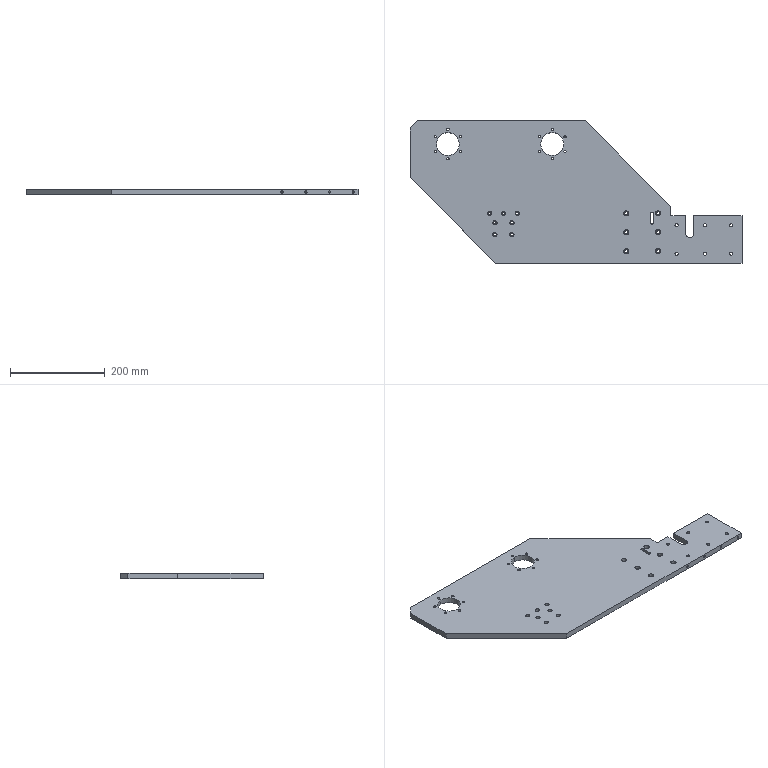Component | SolidWorks | LD101-02--Q1012-Q1-2-5 | 1 solid | 176 faces | box 700 x 300 x 12 mm | volume 1696516 mm3 | cylinder 125 | plane 35 | cone 16 | commonest cylinder face diameters 5 x32 11 x24 6.6 x24 5.5 x17 9 x14 4.2 x8 48.2 x4 17 x2 | material AL6061
build123d program:
from build123d import *

# Parameters (mm, degrees)
SKETCH1_W                                           = 700
SKETCH1_H                                           = 300
BOSS_EXTRUDE1_DEPTH                                 = 6
SKETCH2_W                                           = 150
SKETCH2_H                                           = 200
CUT_EXTRUDE1_DEPTH                                  = 381.978
CUT_EXTRUDE4_DEPTH                                  = 381.978
HOLE_SIZE_ACCORDING_TO_TYPE0_OF_HEXAGON_D           = 6.6
HOLE_SIZE_ACCORDING_TO_TYPE0_OF_HEXAGON_CBORE_D     = 11
HOLE_SIZE_ACCORDING_TO_TYPE0_OF_HEXAGON_CBORE_DEPTH = 6.8
M6_TAPPED_HOLE2_D                                   = 5
M6_TAPPED_HOLE2_DEPTH                               = 20
M6_TAPPED_HOLE2_TIP                                 = 1.502
CUT_EXTRUDE6_DEPTH                                  = 381.978
CUT_EXTRUDE7_DEPTH                                  = 381.978
HOLE_SIZE_FOR_HEX_SOCKET_HEAD_CAP_SCRE_D            = 6.6
HOLE_SIZE_FOR_HEX_SOCKET_HEAD_CAP_SCRE_CBORE_D      = 11
HOLE_SIZE_FOR_HEX_SOCKET_HEAD_CAP_SCRE_CBORE_DEPTH  = 6.8
CHAMFER1_SIZE                                       = 15
SKETCH18_R                                          = 24.1
CUT_EXTRUDE8_DEPTH                                  = 381.978
HOLE_SIZE_ACCORDING_TO_HEXAGON_SOCKET_H_D           = 5.5
HOLE_SIZE_ACCORDING_TO_HEXAGON_SOCKET_H_CBORE_D     = 9
HOLE_SIZE_ACCORDING_TO_HEXAGON_SOCKET_H_CBORE_DEPTH = 5.7
M5_TAPPED_HOLE1_D                                   = 4.2
M5_TAPPED_HOLE1_DEPTH                               = 16
M5_TAPPED_HOLE1_TIP                                 = 1.262
M6_TAPPED_HOLE3_D                                   = 5


with BuildPart() as part:
    # Sketch1 → Boss-Extrude1 (new, symmetric)
    with BuildSketch(Plane(origin=(0, 0, 0), x_dir=(1, 0, 0), z_dir=(0, 1, 0))):
        Rectangle(SKETCH1_W, SKETCH1_H)
    extrude(amount=BOSS_EXTRUDE1_DEPTH, both=True)

    # Sketch2 → Cut-Extrude1 (cut, through all)
    with BuildSketch(Plane.XZ.offset(6)):
        with Locations((275, 50)):
            Rectangle(SKETCH2_W, SKETCH2_H)
    extrude(amount=-CUT_EXTRUDE1_DEPTH, mode=Mode.SUBTRACT)

    # Sketch5 → Cut-Extrude4 (cut, through all)
    with BuildSketch(Plane.XZ.offset(6)):
        with BuildLine():
            Line((157.25, -65), (157.25, -45))
            ThreePointArc((157.25, -45), (160, -42.25), (162.75, -45))
            Line((162.75, -45), (162.75, -65))
            ThreePointArc((162.75, -65), (160, -67.75), (157.25, -65))
        make_face()
    extrude(amount=-CUT_EXTRUDE4_DEPTH, mode=Mode.SUBTRACT)

    # Hole Size_according to_Type0 of Hexagon (through all)
    with Locations(Plane(origin=(0, 6, 0), x_dir=(1, 0, 0), z_dir=(0, 1, 0))):
        with Locations((327, 70), (272, 70), (212, 70), (212, 130), (327, 130), (272, 130)):
            CounterBoreHole(HOLE_SIZE_ACCORDING_TO_TYPE0_OF_HEXAGON_D / 2, HOLE_SIZE_ACCORDING_TO_TYPE0_OF_HEXAGON_CBORE_D / 2, HOLE_SIZE_ACCORDING_TO_TYPE0_OF_HEXAGON_CBORE_DEPTH)

    # M6 Tapped Hole2
    with Locations(Plane(origin=(0, 0, -150), x_dir=(-1, 0, 0), z_dir=(0, 0, -1))):
        with Locations((-340, 0), (-290, 0), (-240, 0), (-190, 0)):
            Hole(M6_TAPPED_HOLE2_D / 2, depth=M6_TAPPED_HOLE2_DEPTH)
            with Locations((0, 0, -(M6_TAPPED_HOLE2_DEPTH + M6_TAPPED_HOLE2_TIP / 2))):  # 118° drill point
                Cone(0, M6_TAPPED_HOLE2_D / 2, M6_TAPPED_HOLE2_TIP, mode=Mode.SUBTRACT)

    # Sketch15 → Cut-Extrude6 (cut, through all)
    with BuildSketch(Plane.XZ.offset(6)):
        with BuildLine():
            Line((248.5, -50), (248.5, -88))
            ThreePointArc((248.5, -88), (240, -96.5), (231.5, -88))
            Line((231.5, -88), (231.5, -50))
            ThreePointArc((231.5, -50), (240, -41.5), (248.5, -50))
        make_face()
    extrude(amount=-CUT_EXTRUDE6_DEPTH, mode=Mode.SUBTRACT)

    # Sketch12 → Cut-Extrude7 (cut, through all)
    with BuildSketch(Plane(origin=(0, 6, 0), x_dir=(1, 0, 0), z_dir=(0, 1, 0))):
        Polygon((-170, 150), (-350, -30), (-350, 150), align=None)
        Polygon((200, -150), (200, 30), (20, -150), align=None)
    extrude(amount=-CUT_EXTRUDE7_DEPTH, mode=Mode.SUBTRACT)

    # Hole Size _for_ Hex Socket Head Cap Scre (through all)
    with Locations(Plane(origin=(0, -6, 0), x_dir=(-1, 0, 0), z_dir=(0, -1, 0))):
        with Locations((-106, 45), (-106, 85), (-106, 125), (-173, 45), (-173, 85), (-173, 125)):
            CounterBoreHole(HOLE_SIZE_FOR_HEX_SOCKET_HEAD_CAP_SCRE_D / 2, HOLE_SIZE_FOR_HEX_SOCKET_HEAD_CAP_SCRE_CBORE_D / 2, HOLE_SIZE_FOR_HEX_SOCKET_HEAD_CAP_SCRE_CBORE_DEPTH)

    # Chamfer1
    chamfer1_edges = [part.edges().sort_by_distance(p)[0] for p in [
        (-350, 0, 150),
    ]]
    chamfer(chamfer1_edges, length=CHAMFER1_SIZE)

    # Sketch18 → Cut-Extrude8 (cut, through all)
    with BuildSketch(Plane.XZ.offset(6)):
        with Locations(Location((-270, 101, 0), (0, 0, 270))):
            Circle(SKETCH18_R)
        with Locations(Location((-50, 101, 0), (0, 0, 270))):
            Circle(SKETCH18_R)
    extrude(amount=-CUT_EXTRUDE8_DEPTH, mode=Mode.SUBTRACT)

    # Hole Size_ according to_Hexagon Socket H (through all)
    with Locations(Plane(origin=(0, -6, 0), x_dir=(-1, 0, 0), z_dir=(0, -1, 0))):
        with Locations((182, 45), (153, 45), (124, 45), (135, 90), (171, 90), (171, 65), (135, 65)):
            CounterBoreHole(HOLE_SIZE_ACCORDING_TO_HEXAGON_SOCKET_H_D / 2, HOLE_SIZE_ACCORDING_TO_HEXAGON_SOCKET_H_CBORE_D / 2, HOLE_SIZE_ACCORDING_TO_HEXAGON_SOCKET_H_CBORE_DEPTH)

    # M5 Tapped Hole1
    with Locations(Plane.XY.offset(150)):
        with Locations((-295, 0), (-205, 0), (-115, 0), (-25, 0)):
            Hole(M5_TAPPED_HOLE1_D / 2, depth=M5_TAPPED_HOLE1_DEPTH)
            with Locations((0, 0, -(M5_TAPPED_HOLE1_DEPTH + M5_TAPPED_HOLE1_TIP / 2))):  # 118° drill point
                Cone(0, M5_TAPPED_HOLE1_D / 2, M5_TAPPED_HOLE1_TIP, mode=Mode.SUBTRACT)

    # M6 Tapped Hole3 (through all)
    with Locations(Plane(origin=(0, 6, 0), x_dir=(1, 0, 0), z_dir=(0, 1, 0))):
        with Locations((-50, -132), (-23.153, -116.5), (-23.153, -85.5), (-50, -70), (-76.847, -85.5), (-76.847, -116.5), (-270, -70), (-243.153, -85.5), (-243.153, -116.5), (-270, -132), (-296.847, -116.5), (-296.847, -85.5)):
            Hole(M6_TAPPED_HOLE3_D / 2)


solid = part.part

# Placed as in the assembly
solid = solid.moved(Location((-600.29, -89.897, -6.743), (-90, 0, 0)))